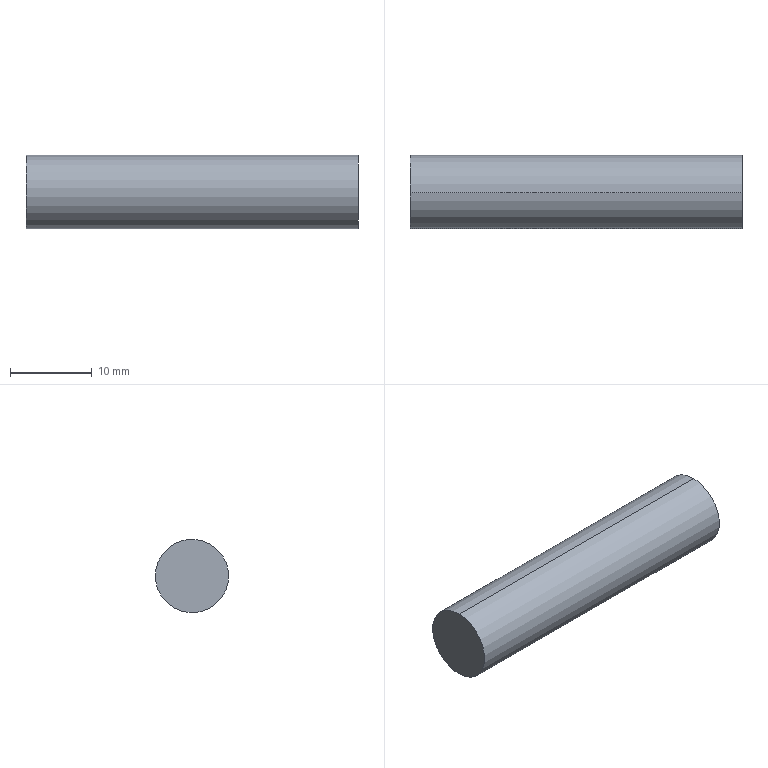Component | SolidWorks | Part5-1 | 1 solid | 4 faces | box 40.71 x 9 x 9 mm | volume 2590 mm3 | cylinder 2 | plane 2 | commonest cylinder face diameters 9 x2 | material 45
build123d program:
from build123d import *

# Parameters (mm, degrees)
SKETCH2_W = 4.5
SKETCH2_H = 40.705


with BuildPart() as part:
    # Sketch2 → Revolve1 (revolve)
    with BuildSketch(Plane.XY, mode=Mode.PRIVATE) as revolve1_sk:
        with Locations((18.75, 15.647)):
            Rectangle(SKETCH2_W, SKETCH2_H)
    revolve(revolve1_sk.sketch.rotate(Axis((16.5, 36, 0), (0, -1, 0)), 90), axis=Axis((16.5, 36, 0), (0, -1, 0)))


solid = part.part

# Placed as in the assembly
solid = solid.moved(Location((6.703, -61.5, 10.004), (0, 0, 90)))
STEP:
#1=CARTESIAN_POINT('',(0.4491,-1.768,0.2167));
#2=VERTEX_POINT('',#1);
#3=CARTESIAN_POINT('',(0.4491,-1.775,0.571));
#4=VERTEX_POINT('',#3);
#5=CARTESIAN_POINT('',(0.4491,-1.772,0.3939));
#6=DIRECTION('',(-1.,-0.,0.));
#7=DIRECTION('',(0.,0.02089,-0.9998));
#8=AXIS2_PLACEMENT_3D('',#5,#6,#7);
#9=CIRCLE('',#8,0.1772);
#10=EDGE_CURVE('',#2,#4,#9,.T.);
#11=ORIENTED_EDGE('',*,*,#10,.T.);
#12=CARTESIAN_POINT('',(-1.153,-1.775,0.571));
#13=VERTEX_POINT('',#12);
#14=CARTESIAN_POINT('',(-1.153,-1.775,0.571));
#15=DIRECTION('',(-1.,-0.,0.));
#16=VECTOR('',#15,39.37);
#17=LINE('',#14,#16);
#18=EDGE_CURVE('',#4,#13,#17,.T.);
#19=ORIENTED_EDGE('',*,*,#18,.T.);
#20=CARTESIAN_POINT('',(-1.153,-1.768,0.2167));
#21=VERTEX_POINT('',#20);
#22=CARTESIAN_POINT('',(-1.153,-1.772,0.3939));
#23=DIRECTION('',(-1.,-0.,0.));
#24=DIRECTION('',(0.,0.02089,-0.9998));
#25=AXIS2_PLACEMENT_3D('',#22,#23,#24);
#26=CIRCLE('',#25,0.1772);
#27=EDGE_CURVE('',#21,#13,#26,.T.);
#28=ORIENTED_EDGE('',*,*,#27,.F.);
#29=CARTESIAN_POINT('',(-1.153,-1.768,0.2167));
#30=DIRECTION('',(-1.,-0.,0.));
#31=VECTOR('',#30,39.37);
#32=LINE('',#29,#31);
#33=EDGE_CURVE('',#2,#21,#32,.T.);
#34=ORIENTED_EDGE('',*,*,#33,.F.);
#35=EDGE_LOOP('',(#11,#19,#28,#34));
#36=FACE_OUTER_BOUND('',#35,.T.);
#37=CARTESIAN_POINT('',(-1.153,-1.772,0.3939));
#38=DIRECTION('',(-1.,-0.,0.));
#39=DIRECTION('',(0.,0.02089,-0.9998));
#40=AXIS2_PLACEMENT_3D('',#37,#38,#39);
#41=CYLINDRICAL_SURFACE('',#40,0.1772);
#42=ADVANCED_FACE('',(#36),#41,.T.);
#43=ORIENTED_EDGE('',*,*,#27,.T.);
#44=CARTESIAN_POINT('',(-1.153,-1.772,0.3939));
#45=DIRECTION('',(-1.,-0.,0.));
#46=DIRECTION('',(0.,0.02089,-0.9998));
#47=AXIS2_PLACEMENT_3D('',#44,#45,#46);
#48=CIRCLE('',#47,0.1772);
#49=EDGE_CURVE('',#13,#21,#48,.T.);
#50=ORIENTED_EDGE('',*,*,#49,.T.);
#51=EDGE_LOOP('',(#43,#50));
#52=FACE_OUTER_BOUND('',#51,.T.);
#53=CARTESIAN_POINT('',(-1.153,-1.772,0.3939));
#54=DIRECTION('',(1.,0.,-0.));
#55=DIRECTION('',(0.,-0.02089,0.9998));
#56=AXIS2_PLACEMENT_3D('',#53,#54,#55);
#57=PLANE('',#56);
#58=ADVANCED_FACE('',(#52),#57,.F.);
#59=ORIENTED_EDGE('',*,*,#18,.F.);
#60=CARTESIAN_POINT('',(0.4491,-1.772,0.3939));
#61=DIRECTION('',(-1.,-0.,0.));
#62=DIRECTION('',(0.,0.02089,-0.9998));
#63=AXIS2_PLACEMENT_3D('',#60,#61,#62);
#64=CIRCLE('',#63,0.1772);
#65=EDGE_CURVE('',#4,#2,#64,.T.);
#66=ORIENTED_EDGE('',*,*,#65,.T.);
#67=ORIENTED_EDGE('',*,*,#33,.T.);
#68=ORIENTED_EDGE('',*,*,#49,.F.);
#69=EDGE_LOOP('',(#59,#66,#67,#68));
#70=FACE_OUTER_BOUND('',#69,.T.);
#71=CARTESIAN_POINT('',(-1.153,-1.772,0.3939));
#72=DIRECTION('',(-1.,-0.,0.));
#73=DIRECTION('',(0.,0.02089,-0.9998));
#74=AXIS2_PLACEMENT_3D('',#71,#72,#73);
#75=CYLINDRICAL_SURFACE('',#74,0.1772);
#76=ADVANCED_FACE('',(#70),#75,.T.);
#77=ORIENTED_EDGE('',*,*,#10,.F.);
#78=ORIENTED_EDGE('',*,*,#65,.F.);
#79=EDGE_LOOP('',(#77,#78));
#80=FACE_OUTER_BOUND('',#79,.T.);
#81=CARTESIAN_POINT('',(0.4491,-1.949,0.3902));
#82=DIRECTION('',(-1.,-0.,0.));
#83=DIRECTION('',(-0.,0.02089,-0.9998));
#84=AXIS2_PLACEMENT_3D('',#81,#82,#83);
#85=PLANE('',#84);
#86=ADVANCED_FACE('',(#80),#85,.F.);
#87=CLOSED_SHELL('',(#42,#58,#76,#86));
#88=MANIFOLD_SOLID_BREP('',#87);
#89=CARTESIAN_POINT('',(0.,0.,0.));
#90=DIRECTION('',(0.,0.,1.));
#91=DIRECTION('',(1.,0.,0.));
#92=AXIS2_PLACEMENT_3D('',#89,#90,#91);
#93=(LENGTH_UNIT()NAMED_UNIT(*)SI_UNIT($,.METRE.));
#94=LENGTH_MEASURE_WITH_UNIT(LENGTH_MEASURE(0.0254),#93);
#95=DIMENSIONAL_EXPONENTS(1.,0.,0.,0.,0.,0.,0.);
#96=(CONVERSION_BASED_UNIT('',#94)LENGTH_UNIT()NAMED_UNIT(#95));
#97=UNCERTAINTY_MEASURE_WITH_UNIT(LENGTH_MEASURE(0.00001),#96,'','');
#98=(NAMED_UNIT(*)PLANE_ANGLE_UNIT()SI_UNIT($,.RADIAN.));
#99=(NAMED_UNIT(*)SI_UNIT($,.STERADIAN.)SOLID_ANGLE_UNIT());
#100=(GEOMETRIC_REPRESENTATION_CONTEXT(3)GLOBAL_UNCERTAINTY_ASSIGNED_CONTEXT((#97))GLOBAL_UNIT_ASSIGNED_CONTEXT((#96,#98,#99))REPRESENTATION_CONTEXT('',''));
#101=ADVANCED_BREP_SHAPE_REPRESENTATION('',(#88,#92),#100);
#102=COLOUR_RGB('',0.7922,0.8196,0.9333);
#103=FILL_AREA_STYLE_COLOUR('',#102);
#104=FILL_AREA_STYLE('',(#103));
#105=SURFACE_STYLE_FILL_AREA(#104);
#106=SURFACE_SIDE_STYLE('',(#105));
#107=SURFACE_STYLE_USAGE(.BOTH.,#106);
#108=PRESENTATION_STYLE_ASSIGNMENT((#107));
#109=STYLED_ITEM('',(#108),#88);
#110=(LENGTH_UNIT()NAMED_UNIT(*)SI_UNIT($,.METRE.));
#111=LENGTH_MEASURE_WITH_UNIT(LENGTH_MEASURE(0.0254),#110);
#112=DIMENSIONAL_EXPONENTS(1.,0.,0.,0.,0.,0.,0.);
#113=(CONVERSION_BASED_UNIT('',#111)LENGTH_UNIT()NAMED_UNIT(#112));
#114=UNCERTAINTY_MEASURE_WITH_UNIT(LENGTH_MEASURE(0.00001),#113,'','');
#115=(NAMED_UNIT(*)PLANE_ANGLE_UNIT()SI_UNIT($,.RADIAN.));
#116=(NAMED_UNIT(*)SI_UNIT($,.STERADIAN.)SOLID_ANGLE_UNIT());
#117=(GEOMETRIC_REPRESENTATION_CONTEXT(3)GLOBAL_UNCERTAINTY_ASSIGNED_CONTEXT((#114))GLOBAL_UNIT_ASSIGNED_CONTEXT((#113,#115,#116))REPRESENTATION_CONTEXT('',''));
#118=MECHANICAL_DESIGN_GEOMETRIC_PRESENTATION_REPRESENTATION('',(#109),#117);
#119=PRESENTATION_LAYER_ASSIGNMENT('','',(#109));